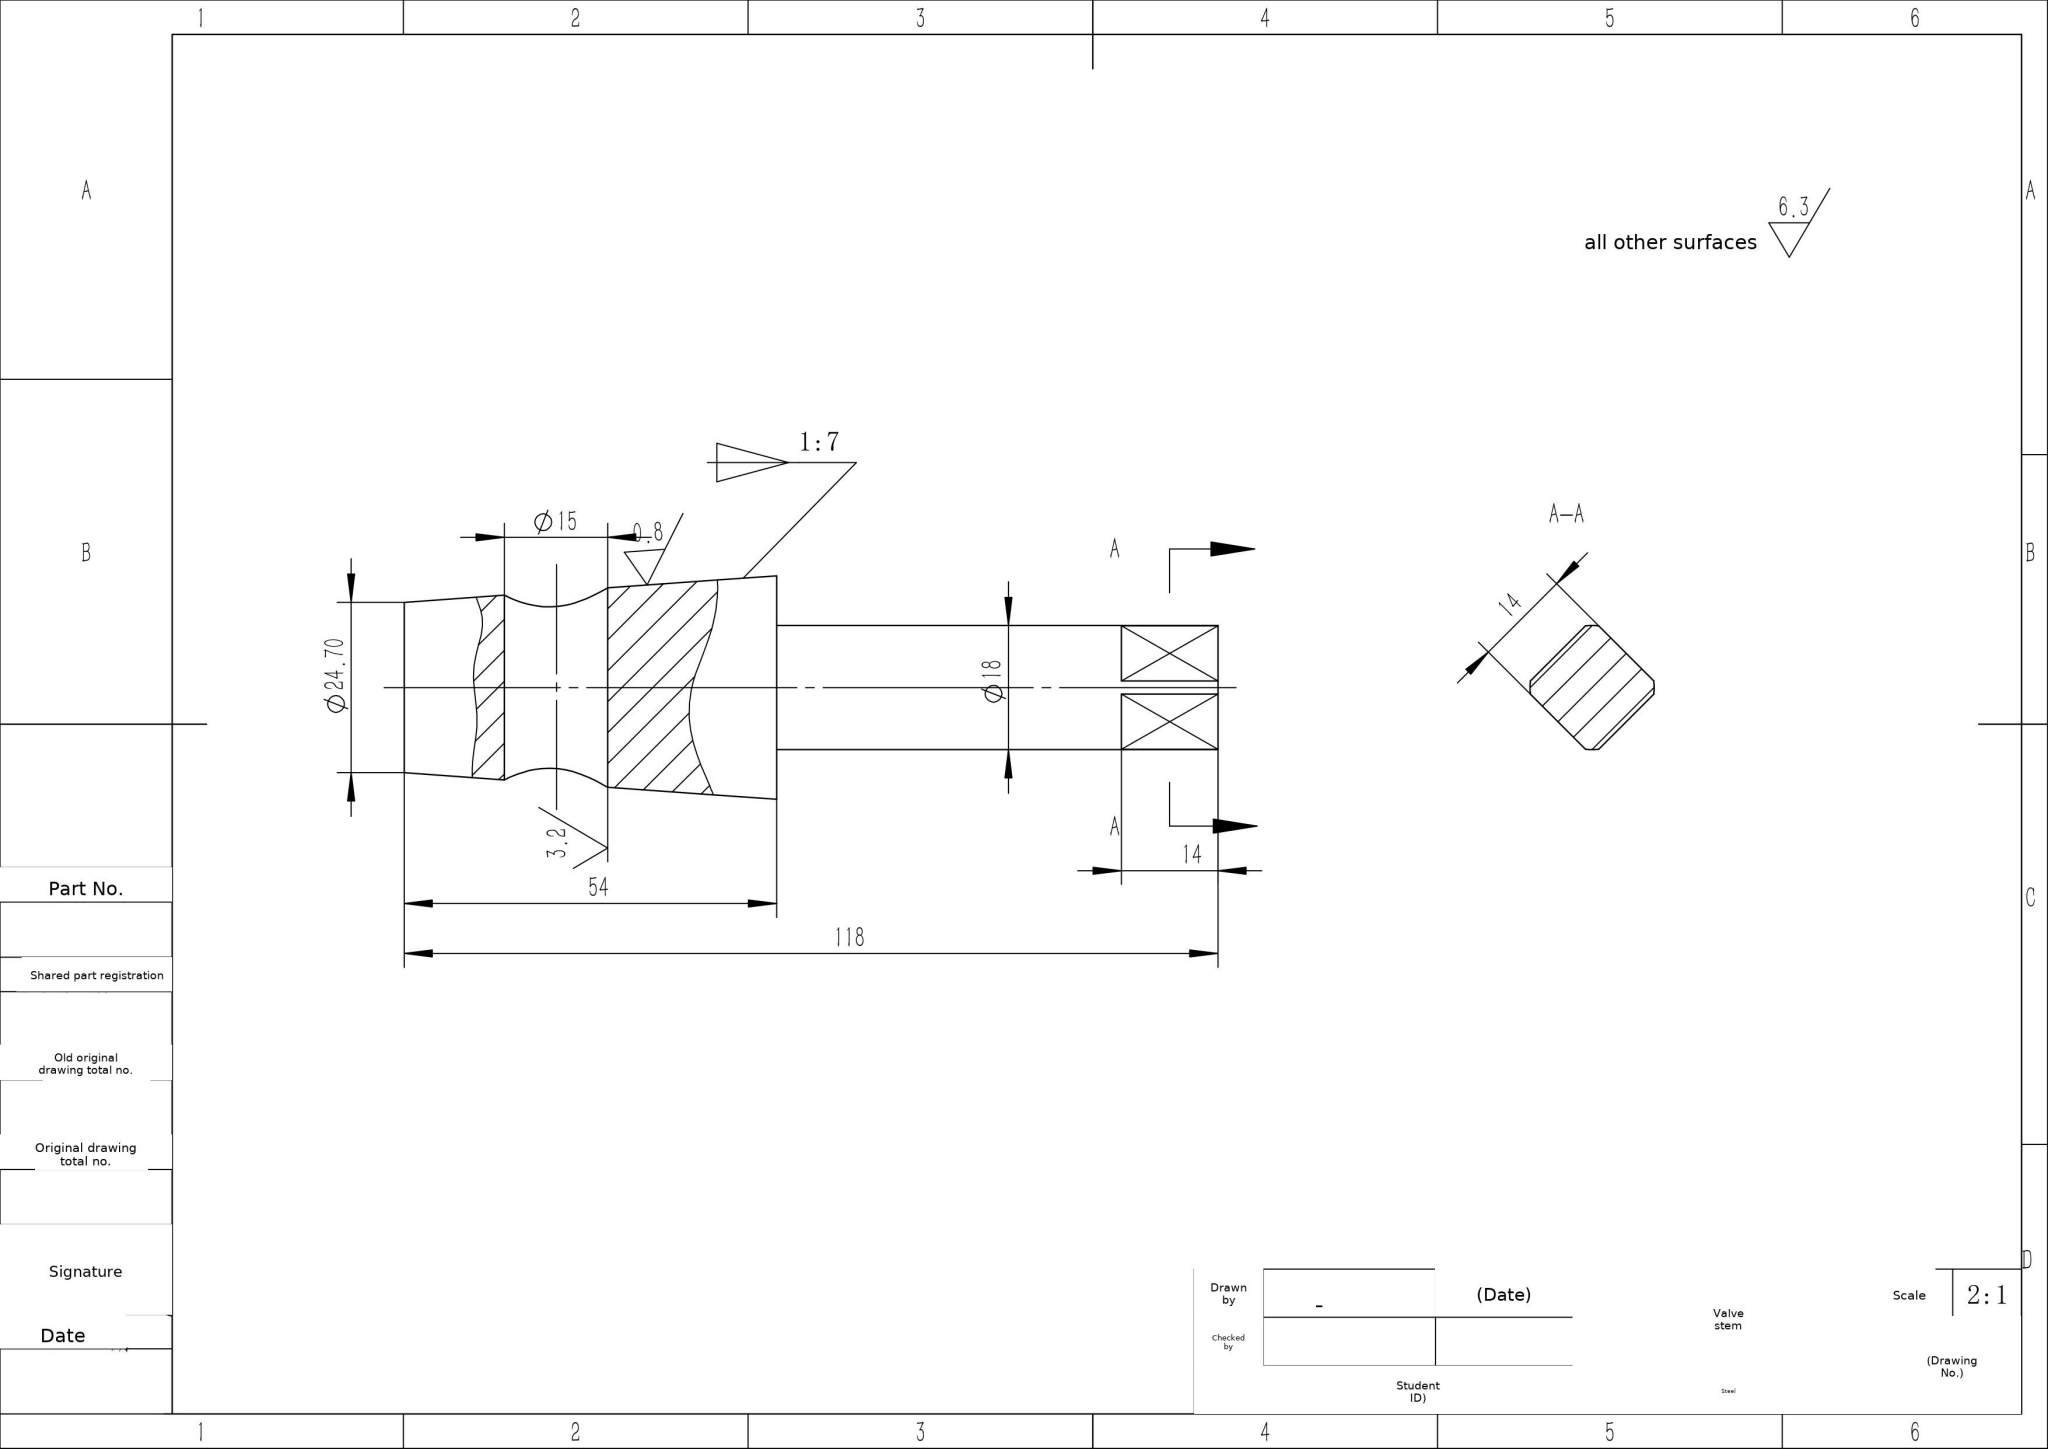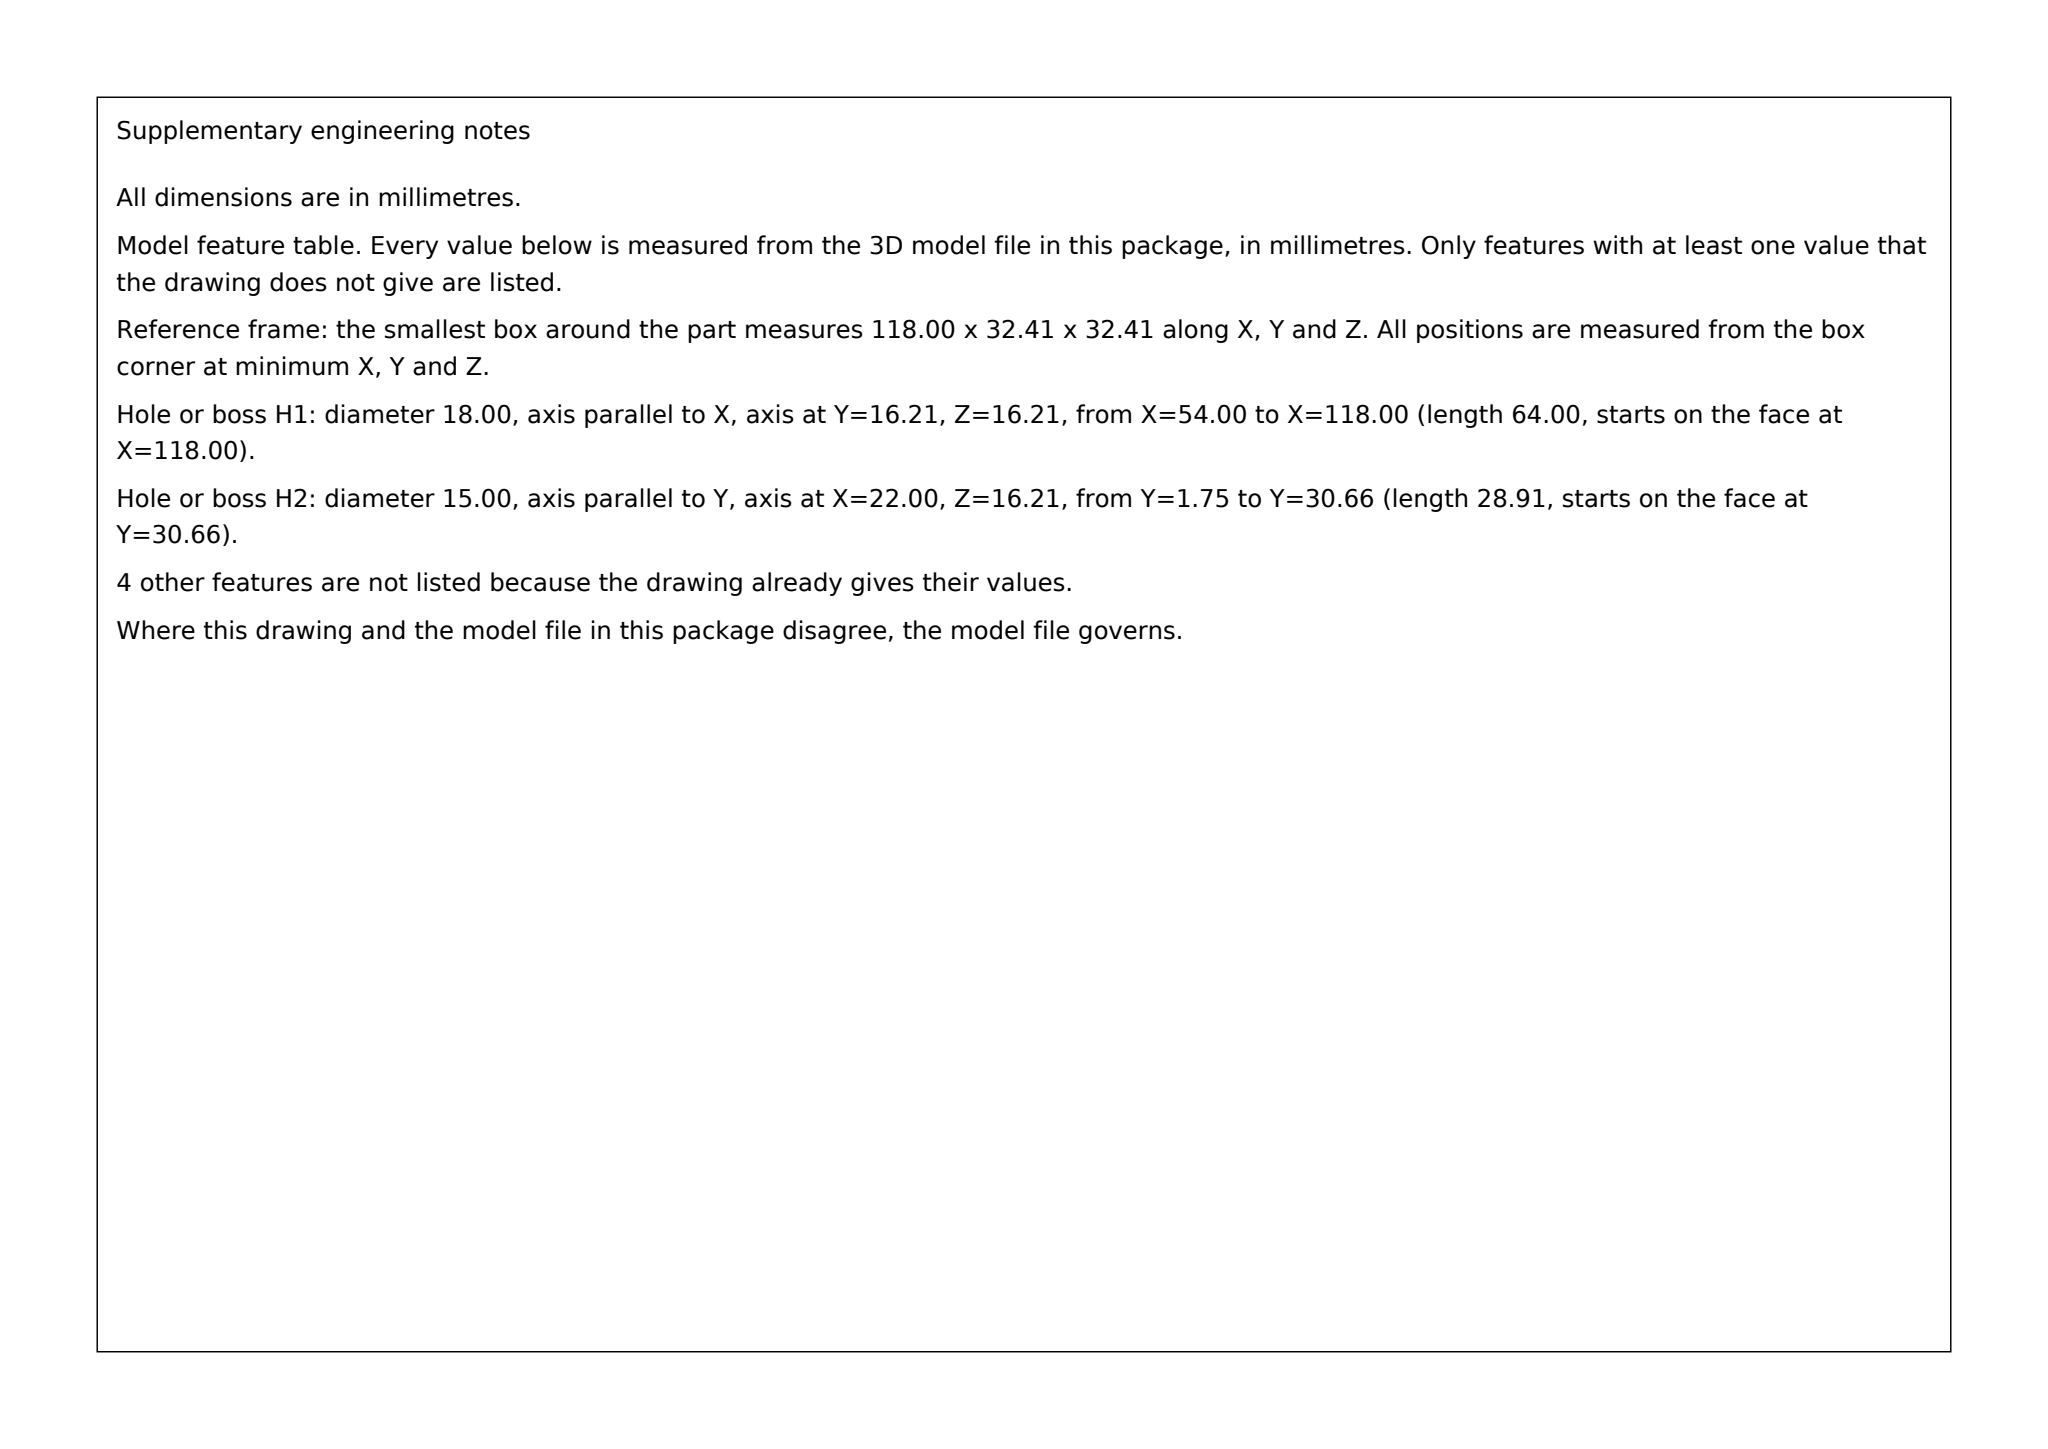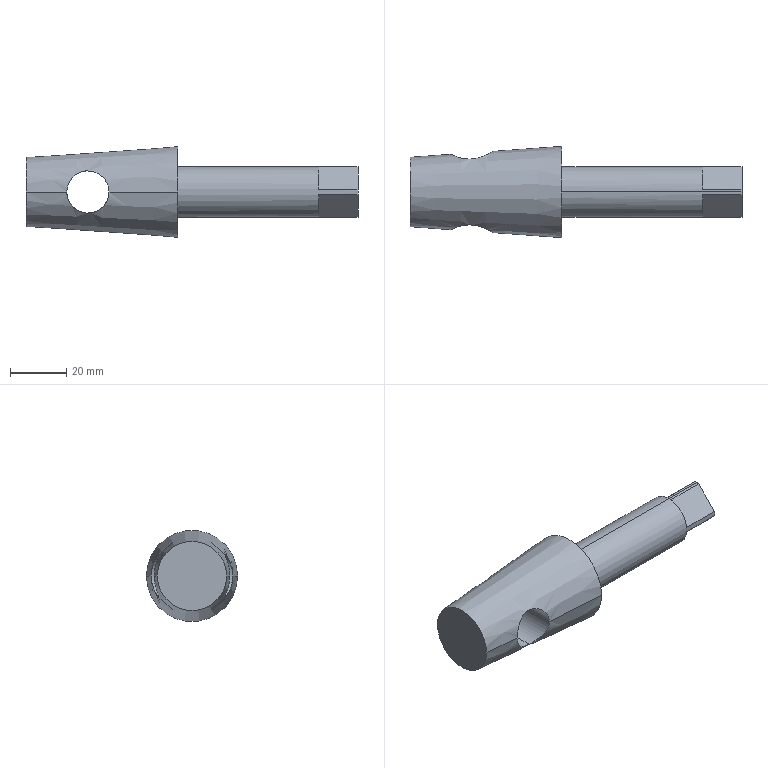Part | SolidWorks | mm | material Steel | 1 solid | 17 faces | box 118 x 32.41 x 32.41 mm | volume 45483 mm3 | plane 11 | cylinder 4 | cone 2 | commonest cylinder face diameters 15 x2 18 x2
build123d program:
from build123d import *

# Parameters (mm, degrees)
SKETCH2_R           = 9
BOSS_EXTRUDE1_DEPTH = 64
SKETCH5_R           = 7.5
CUT_EXTRUDE1_DEPTH  = 32
CUT_EXTRUDE2_DEPTH  = 14


with BuildPart() as part:
    # Sketch2 → Boss-Extrude1 (new body)
    with BuildSketch(Plane(origin=(0, 0, 0), x_dir=(0, 0, -1), z_dir=(1, 0, 0))):
        Circle(SKETCH2_R)
    extrude(amount=BOSS_EXTRUDE1_DEPTH)

    # Sketch3 → Revolve2 (revolve)
    with BuildSketch(Plane.XY, mode=Mode.PRIVATE) as revolve2_sk:
        Polygon((0, 0), (0, 16.207), (-54, 12.35), (-54, 0), align=None)
    revolve(revolve2_sk.sketch.rotate(Axis((-54, 0, 0), (1, 0, 0)), 180), axis=Axis((-54, 0, 0), (1, 0, 0)))

    # Sketch5 → Cut-Extrude1 (cut, symmetric)
    with BuildSketch(Plane(origin=(0, 0, 0), x_dir=(1, 0, 0), z_dir=(0, 1, 0))):
        with Locations(Location((-32, 0, 0), (0, 0, 180))):
            Circle(SKETCH5_R)
    extrude(amount=CUT_EXTRUDE1_DEPTH, both=True, mode=Mode.SUBTRACT)

    # Sketch6 → Cut-Extrude2 (cut)
    with BuildSketch(Plane(origin=(64, 0, 0), x_dir=(0, 0, -1), z_dir=(1, 0, 0))):
        Polygon((-24.042, 0), (0, 24.042), (24.042, 0), (0, -24.042), align=None)
        Polygon((0, -9.899), (9.899, 0), (0, 9.899), (-9.899, 0), align=None, mode=Mode.SUBTRACT)
    extrude(amount=-CUT_EXTRUDE2_DEPTH, mode=Mode.SUBTRACT)


solid = part.part
STEP:
#1=CARTESIAN_POINT('',(-32.,-11.728,-7.5));
#2=VERTEX_POINT('',#1);
#3=CARTESIAN_POINT('',(-39.5,-13.386,0.));
#4=VERTEX_POINT('',#3);
#5=CARTESIAN_POINT('',(-32.,-11.728,-7.5));
#6=CARTESIAN_POINT('',(-32.498,-11.686,-7.5));
#7=CARTESIAN_POINT('',(-32.991,-11.676,-7.451));
#8=CARTESIAN_POINT('',(-33.722,-11.707,-7.304));
#9=CARTESIAN_POINT('',(-33.965,-11.725,-7.242));
#10=CARTESIAN_POINT('',(-34.442,-11.774,-7.096));
#11=CARTESIAN_POINT('',(-34.674,-11.806,-7.011));
#12=CARTESIAN_POINT('',(-35.127,-11.879,-6.821));
#13=CARTESIAN_POINT('',(-35.348,-11.921,-6.716));
#14=CARTESIAN_POINT('',(-35.78,-12.015,-6.483));
#15=CARTESIAN_POINT('',(-35.991,-12.066,-6.355));
#16=CARTESIAN_POINT('',(-36.598,-12.227,-5.945));
#17=CARTESIAN_POINT('',(-36.972,-12.345,-5.636));
#18=CARTESIAN_POINT('',(-37.658,-12.585,-4.947));
#19=CARTESIAN_POINT('',(-37.965,-12.704,-4.572));
#20=CARTESIAN_POINT('',(-38.367,-12.87,-3.971));
#21=CARTESIAN_POINT('',(-38.492,-12.923,-3.764));
#22=CARTESIAN_POINT('',(-38.722,-13.023,-3.335));
#23=CARTESIAN_POINT('',(-38.828,-13.07,-3.112));
#24=CARTESIAN_POINT('',(-39.112,-13.199,-2.432));
#25=CARTESIAN_POINT('',(-39.255,-13.267,-1.964));
#26=CARTESIAN_POINT('',(-39.449,-13.361,-0.9992));
#27=CARTESIAN_POINT('',(-39.5,-13.386,-0.4958));
#28=CARTESIAN_POINT('',(-39.5,-13.386,0.));
#29=B_SPLINE_CURVE_WITH_KNOTS('',3,(#5,#6,#7,#8,#9,#10,#11,#12,#13,#14,#15,#16,#17,#18,#19,#20,#21,#22,#23,#24,#25,#26,#27,#28),.UNSPECIFIED.,.F.,.F.,(4,2,2,2,2,2,2,2,2,2,2,4),(0.04176,0.04324,0.04398,0.04472,0.04547,0.04621,0.04769,0.04917,0.04992,0.05066,0.05214,0.05363),.UNSPECIFIED.);
#30=EDGE_CURVE('',#2,#4,#29,.T.);
#31=ORIENTED_EDGE('',*,*,#30,.F.);
#32=CARTESIAN_POINT('',(-32.,11.728,-7.5));
#33=VERTEX_POINT('',#32);
#34=CARTESIAN_POINT('',(-32.,-32.,-7.5));
#35=DIRECTION('',(0.,1.,0.));
#36=VECTOR('',#35,1000.);
#37=LINE('',#34,#36);
#38=EDGE_CURVE('',#2,#33,#37,.T.);
#39=ORIENTED_EDGE('',*,*,#38,.T.);
#40=CARTESIAN_POINT('',(-39.5,13.386,0.));
#41=VERTEX_POINT('',#40);
#42=CARTESIAN_POINT('',(-39.5,13.386,0.));
#43=CARTESIAN_POINT('',(-39.5,13.386,-0.5028));
#44=CARTESIAN_POINT('',(-39.45,13.361,-0.9965));
#45=CARTESIAN_POINT('',(-39.255,13.267,-1.965));
#46=CARTESIAN_POINT('',(-39.107,13.197,-2.445));
#47=CARTESIAN_POINT('',(-38.729,13.025,-3.349));
#48=CARTESIAN_POINT('',(-38.498,12.923,-3.777));
#49=CARTESIAN_POINT('',(-37.954,12.7,-4.587));
#50=CARTESIAN_POINT('',(-37.644,12.579,-4.963));
#51=CARTESIAN_POINT('',(-37.129,12.4,-5.478));
#52=CARTESIAN_POINT('',(-36.948,12.34,-5.642));
#53=CARTESIAN_POINT('',(-36.573,12.225,-5.949));
#54=CARTESIAN_POINT('',(-36.379,12.169,-6.093));
#55=CARTESIAN_POINT('',(-35.778,12.01,-6.497));
#56=CARTESIAN_POINT('',(-35.348,11.915,-6.73));
#57=CARTESIAN_POINT('',(-34.435,11.767,-7.111));
#58=CARTESIAN_POINT('',(-33.965,11.717,-7.255));
#59=CARTESIAN_POINT('',(-33.24,11.687,-7.401));
#60=CARTESIAN_POINT('',(-32.995,11.684,-7.438));
#61=CARTESIAN_POINT('',(-32.497,11.694,-7.488));
#62=CARTESIAN_POINT('',(-32.247,11.707,-7.5));
#63=CARTESIAN_POINT('',(-32.,11.728,-7.5));
#64=B_SPLINE_CURVE_WITH_KNOTS('',3,(#42,#43,#44,#45,#46,#47,#48,#49,#50,#51,#52,#53,#54,#55,#56,#57,#58,#59,#60,#61,#62,#63),.UNSPECIFIED.,.F.,.F.,(4,2,2,2,2,2,2,2,2,2,4),(0.04154,0.04302,0.04451,0.04599,0.04747,0.04822,0.04896,0.05044,0.05192,0.05267,0.05341),.UNSPECIFIED.);
#65=EDGE_CURVE('',#41,#33,#64,.T.);
#66=ORIENTED_EDGE('',*,*,#65,.F.);
#67=CARTESIAN_POINT('',(-32.,11.728,7.5));
#68=VERTEX_POINT('',#67);
#69=CARTESIAN_POINT('',(-32.,11.728,7.5));
#70=CARTESIAN_POINT('',(-32.499,11.686,7.5));
#71=CARTESIAN_POINT('',(-32.991,11.676,7.451));
#72=CARTESIAN_POINT('',(-33.963,11.717,7.255));
#73=CARTESIAN_POINT('',(-34.446,11.769,7.107));
#74=CARTESIAN_POINT('',(-35.353,11.916,6.727));
#75=CARTESIAN_POINT('',(-35.785,12.011,6.493));
#76=CARTESIAN_POINT('',(-36.597,12.227,5.946));
#77=CARTESIAN_POINT('',(-36.969,12.344,5.639));
#78=CARTESIAN_POINT('',(-37.651,12.582,4.955));
#79=CARTESIAN_POINT('',(-37.963,12.703,4.575));
#80=CARTESIAN_POINT('',(-38.501,12.925,3.771));
#81=CARTESIAN_POINT('',(-38.731,13.026,3.345));
#82=CARTESIAN_POINT('',(-39.015,13.155,2.666));
#83=CARTESIAN_POINT('',(-39.099,13.194,2.431));
#84=CARTESIAN_POINT('',(-39.244,13.262,1.958));
#85=CARTESIAN_POINT('',(-39.304,13.291,1.719));
#86=CARTESIAN_POINT('',(-39.45,13.361,0.9954));
#87=CARTESIAN_POINT('',(-39.5,13.386,0.503));
#88=CARTESIAN_POINT('',(-39.5,13.386,0.));
#89=B_SPLINE_CURVE_WITH_KNOTS('',3,(#69,#70,#71,#72,#73,#74,#75,#76,#77,#78,#79,#80,#81,#82,#83,#84,#85,#86,#87,#88),.UNSPECIFIED.,.F.,.F.,(4,2,2,2,2,2,2,2,2,4),(0.02967,0.03115,0.03264,0.03412,0.0356,0.03709,0.03857,0.03931,0.04006,0.04154),.UNSPECIFIED.);
#90=EDGE_CURVE('',#68,#41,#89,.T.);
#91=ORIENTED_EDGE('',*,*,#90,.F.);
#92=CARTESIAN_POINT('',(-32.,-11.728,7.5));
#93=VERTEX_POINT('',#92);
#94=CARTESIAN_POINT('',(-32.,-32.,7.5));
#95=DIRECTION('',(0.,1.,0.));
#96=VECTOR('',#95,1000.);
#97=LINE('',#94,#96);
#98=EDGE_CURVE('',#93,#68,#97,.T.);
#99=ORIENTED_EDGE('',*,*,#98,.F.);
#100=CARTESIAN_POINT('',(-39.5,-13.386,0.));
#101=CARTESIAN_POINT('',(-39.5,-13.386,0.4967));
#102=CARTESIAN_POINT('',(-39.451,-13.362,0.9892));
#103=CARTESIAN_POINT('',(-39.304,-13.291,1.721));
#104=CARTESIAN_POINT('',(-39.242,-13.262,1.964));
#105=CARTESIAN_POINT('',(-39.098,-13.194,2.436));
#106=CARTESIAN_POINT('',(-39.014,-13.155,2.667));
#107=CARTESIAN_POINT('',(-38.826,-13.069,3.118));
#108=CARTESIAN_POINT('',(-38.721,-13.022,3.338));
#109=CARTESIAN_POINT('',(-38.488,-12.921,3.77));
#110=CARTESIAN_POINT('',(-38.361,-12.867,3.98));
#111=CARTESIAN_POINT('',(-37.955,-12.7,4.585));
#112=CARTESIAN_POINT('',(-37.649,-12.581,4.957));
#113=CARTESIAN_POINT('',(-37.136,-12.403,5.471));
#114=CARTESIAN_POINT('',(-36.955,-12.343,5.636));
#115=CARTESIAN_POINT('',(-36.58,-12.227,5.944));
#116=CARTESIAN_POINT('',(-36.385,-12.171,6.089));
#117=CARTESIAN_POINT('',(-35.784,-12.011,6.494));
#118=CARTESIAN_POINT('',(-35.356,-11.916,6.725));
#119=CARTESIAN_POINT('',(-34.67,-11.805,7.013));
#120=CARTESIAN_POINT('',(-34.436,-11.774,7.098));
#121=CARTESIAN_POINT('',(-33.964,-11.725,7.243));
#122=CARTESIAN_POINT('',(-33.725,-11.707,7.303));
#123=CARTESIAN_POINT('',(-33.241,-11.687,7.401));
#124=CARTESIAN_POINT('',(-32.997,-11.684,7.438));
#125=CARTESIAN_POINT('',(-32.501,-11.694,7.487));
#126=CARTESIAN_POINT('',(-32.249,-11.707,7.5));
#127=CARTESIAN_POINT('',(-32.,-11.728,7.5));
#128=B_SPLINE_CURVE_WITH_KNOTS('',3,(#100,#101,#102,#103,#104,#105,#106,#107,#108,#109,#110,#111,#112,#113,#114,#115,#116,#117,#118,#119,#120,#121,#122,#123,#124,#125,#126,#127),.UNSPECIFIED.,.F.,.F.,(4,2,2,2,2,2,2,2,2,2,2,2,2,4),(0.005728,0.007215,0.007958,0.008701,0.009444,0.01019,0.01167,0.01242,0.01316,0.01465,0.01539,0.01613,0.01688,0.01762),.UNSPECIFIED.);
#129=EDGE_CURVE('',#4,#93,#128,.T.);
#130=ORIENTED_EDGE('',*,*,#129,.F.);
#131=EDGE_LOOP('',(#31,#39,#66,#91,#99,#130));
#132=FACE_OUTER_BOUND('',#131,.T.);
#133=CARTESIAN_POINT('',(-32.,-32.,-0.));
#134=DIRECTION('',(0.,1.,0.));
#135=DIRECTION('',(0.,0.,1.));
#136=AXIS2_PLACEMENT_3D('',#133,#134,#135);
#137=CYLINDRICAL_SURFACE('',#136,7.5);
#138=ADVANCED_FACE('',(#132),#137,.F.);
#139=CARTESIAN_POINT('',(-54.,-12.35,0.));
#140=VERTEX_POINT('',#139);
#141=CARTESIAN_POINT('',(-54.,12.35,0.));
#142=VERTEX_POINT('',#141);
#143=CARTESIAN_POINT('',(-54.,0.,0.));
#144=DIRECTION('',(-1.,0.,0.));
#145=DIRECTION('',(-0.,-1.,0.));
#146=AXIS2_PLACEMENT_3D('',#143,#144,#145);
#147=CIRCLE('',#146,12.35);
#148=EDGE_CURVE('',#140,#142,#147,.T.);
#149=ORIENTED_EDGE('',*,*,#148,.F.);
#150=CARTESIAN_POINT('',(-0.,-16.207,0.));
#151=DIRECTION('',(0.9975,-0.07125,0.));
#152=VECTOR('',#151,1000.);
#153=LINE('',#150,#152);
#154=EDGE_CURVE('',#140,#4,#153,.T.);
#155=ORIENTED_EDGE('',*,*,#154,.T.);
#156=ORIENTED_EDGE('',*,*,#129,.T.);
#157=CARTESIAN_POINT('',(-24.5,-14.457,0.));
#158=VERTEX_POINT('',#157);
#159=CARTESIAN_POINT('',(-32.,-11.728,7.5));
#160=CARTESIAN_POINT('',(-31.494,-11.771,7.5));
#161=CARTESIAN_POINT('',(-30.997,-11.846,7.449));
#162=CARTESIAN_POINT('',(-30.267,-11.999,7.301));
#163=CARTESIAN_POINT('',(-30.025,-12.056,7.239));
#164=CARTESIAN_POINT('',(-29.554,-12.181,7.094));
#165=CARTESIAN_POINT('',(-29.325,-12.248,7.011));
#166=CARTESIAN_POINT('',(-28.878,-12.39,6.824));
#167=CARTESIAN_POINT('',(-28.66,-12.465,6.719));
#168=CARTESIAN_POINT('',(-28.233,-12.62,6.49));
#169=CARTESIAN_POINT('',(-28.025,-12.701,6.365));
#170=CARTESIAN_POINT('',(-27.427,-12.944,5.964));
#171=CARTESIAN_POINT('',(-27.058,-13.109,5.662));
#172=CARTESIAN_POINT('',(-26.377,-13.432,4.986));
#173=CARTESIAN_POINT('',(-26.065,-13.591,4.61));
#174=CARTESIAN_POINT('',(-25.523,-13.876,3.811));
#175=CARTESIAN_POINT('',(-25.289,-14.005,3.385));
#176=CARTESIAN_POINT('',(-24.999,-14.168,2.702));
#177=CARTESIAN_POINT('',(-24.912,-14.218,2.465));
#178=CARTESIAN_POINT('',(-24.764,-14.303,1.988));
#179=CARTESIAN_POINT('',(-24.702,-14.339,1.746));
#180=CARTESIAN_POINT('',(-24.552,-14.426,1.013));
#181=CARTESIAN_POINT('',(-24.5,-14.457,0.5114));
#182=CARTESIAN_POINT('',(-24.5,-14.457,0.));
#183=B_SPLINE_CURVE_WITH_KNOTS('',3,(#159,#160,#161,#162,#163,#164,#165,#166,#167,#168,#169,#170,#171,#172,#173,#174,#175,#176,#177,#178,#179,#180,#181,#182),.UNSPECIFIED.,.F.,.F.,(4,2,2,2,2,2,2,2,2,2,2,4),(0.01762,0.01913,0.01988,0.02064,0.02139,0.02215,0.02366,0.02517,0.02668,0.02744,0.02819,0.0297),.UNSPECIFIED.);
#184=EDGE_CURVE('',#93,#158,#183,.T.);
#185=ORIENTED_EDGE('',*,*,#184,.T.);
#186=CARTESIAN_POINT('',(-0.,-16.207,0.));
#187=VERTEX_POINT('',#186);
#188=CARTESIAN_POINT('',(-0.,-16.207,0.));
#189=DIRECTION('',(0.9975,-0.07125,0.));
#190=VECTOR('',#189,1000.);
#191=LINE('',#188,#190);
#192=EDGE_CURVE('',#158,#187,#191,.T.);
#193=ORIENTED_EDGE('',*,*,#192,.T.);
#194=CARTESIAN_POINT('',(-0.,16.207,0.));
#195=VERTEX_POINT('',#194);
#196=CARTESIAN_POINT('',(-0.,0.,0.));
#197=DIRECTION('',(-1.,0.,0.));
#198=DIRECTION('',(-0.,-1.,0.));
#199=AXIS2_PLACEMENT_3D('',#196,#197,#198);
#200=CIRCLE('',#199,16.207);
#201=EDGE_CURVE('',#187,#195,#200,.T.);
#202=ORIENTED_EDGE('',*,*,#201,.T.);
#203=CARTESIAN_POINT('',(-24.5,14.457,-0.));
#204=VERTEX_POINT('',#203);
#205=CARTESIAN_POINT('',(-0.,16.207,0.));
#206=DIRECTION('',(0.9975,0.07125,0.));
#207=VECTOR('',#206,1000.);
#208=LINE('',#205,#207);
#209=EDGE_CURVE('',#204,#195,#208,.T.);
#210=ORIENTED_EDGE('',*,*,#209,.F.);
#211=CARTESIAN_POINT('',(-24.5,14.457,-0.));
#212=CARTESIAN_POINT('',(-24.5,14.457,0.507));
#213=CARTESIAN_POINT('',(-24.551,14.427,1.007));
#214=CARTESIAN_POINT('',(-24.702,14.339,1.747));
#215=CARTESIAN_POINT('',(-24.765,14.302,1.994));
#216=CARTESIAN_POINT('',(-24.914,14.216,2.471));
#217=CARTESIAN_POINT('',(-25.,14.168,2.704));
#218=CARTESIAN_POINT('',(-25.193,14.059,3.158));
#219=CARTESIAN_POINT('',(-25.3,14.,3.379));
#220=CARTESIAN_POINT('',(-25.536,13.871,3.811));
#221=CARTESIAN_POINT('',(-25.664,13.802,4.021));
#222=CARTESIAN_POINT('',(-26.075,13.586,4.624));
#223=CARTESIAN_POINT('',(-26.382,13.43,4.992));
#224=CARTESIAN_POINT('',(-26.895,13.186,5.5));
#225=CARTESIAN_POINT('',(-27.075,13.103,5.662));
#226=CARTESIAN_POINT('',(-27.447,12.939,5.965));
#227=CARTESIAN_POINT('',(-27.639,12.857,6.107));
#228=CARTESIAN_POINT('',(-28.235,12.616,6.504));
#229=CARTESIAN_POINT('',(-28.657,12.46,6.732));
#230=CARTESIAN_POINT('',(-29.561,12.174,7.109));
#231=CARTESIAN_POINT('',(-30.029,12.048,7.253));
#232=CARTESIAN_POINT('',(-30.751,11.898,7.399));
#233=CARTESIAN_POINT('',(-30.995,11.854,7.437));
#234=CARTESIAN_POINT('',(-31.492,11.78,7.487));
#235=CARTESIAN_POINT('',(-31.746,11.75,7.5));
#236=CARTESIAN_POINT('',(-32.,11.728,7.5));
#237=B_SPLINE_CURVE_WITH_KNOTS('',3,(#211,#212,#213,#214,#215,#216,#217,#218,#219,#220,#221,#222,#223,#224,#225,#226,#227,#228,#229,#230,#231,#232,#233,#234,#235,#236),.UNSPECIFIED.,.F.,.F.,(4,2,2,2,2,2,2,2,2,2,2,2,4),(0.01758,0.01909,0.01985,0.0206,0.02136,0.02211,0.02362,0.02438,0.02514,0.02665,0.02816,0.02891,0.02967),.UNSPECIFIED.);
#238=EDGE_CURVE('',#204,#68,#237,.T.);
#239=ORIENTED_EDGE('',*,*,#238,.T.);
#240=ORIENTED_EDGE('',*,*,#90,.T.);
#241=CARTESIAN_POINT('',(-0.,16.207,0.));
#242=DIRECTION('',(0.9975,0.07125,0.));
#243=VECTOR('',#242,1000.);
#244=LINE('',#241,#243);
#245=EDGE_CURVE('',#142,#41,#244,.T.);
#246=ORIENTED_EDGE('',*,*,#245,.F.);
#247=EDGE_LOOP('',(#149,#155,#156,#185,#193,#202,#210,#239,#240,#246));
#248=FACE_OUTER_BOUND('',#247,.T.);
#249=CARTESIAN_POINT('',(-0.,0.,0.));
#250=DIRECTION('',(1.,-0.,0.));
#251=DIRECTION('',(0.,1.,0.));
#252=AXIS2_PLACEMENT_3D('',#249,#250,#251);
#253=CONICAL_SURFACE('',#252,16.207,0.07131);
#254=ADVANCED_FACE('',(#248),#253,.T.);
#255=CARTESIAN_POINT('',(64.,0.,-9.));
#256=VERTEX_POINT('',#255);
#257=CARTESIAN_POINT('',(64.,0.9497,-8.95));
#258=VERTEX_POINT('',#257);
#259=CARTESIAN_POINT('',(64.,0.,0.));
#260=DIRECTION('',(1.,0.,0.));
#261=DIRECTION('',(0.,0.,-1.));
#262=AXIS2_PLACEMENT_3D('',#259,#260,#261);
#263=CIRCLE('',#262,9.);
#264=EDGE_CURVE('',#256,#258,#263,.T.);
#265=ORIENTED_EDGE('',*,*,#264,.F.);
#266=CARTESIAN_POINT('',(0.,0.,-9.));
#267=VERTEX_POINT('',#266);
#268=CARTESIAN_POINT('',(64.,0.,-9.));
#269=DIRECTION('',(-1.,0.,0.));
#270=VECTOR('',#269,1000.);
#271=LINE('',#268,#270);
#272=EDGE_CURVE('',#256,#267,#271,.T.);
#273=ORIENTED_EDGE('',*,*,#272,.T.);
#274=CARTESIAN_POINT('',(0.,0.,9.));
#275=VERTEX_POINT('',#274);
#276=CARTESIAN_POINT('',(0.,0.,0.));
#277=DIRECTION('',(1.,0.,0.));
#278=DIRECTION('',(0.,0.,-1.));
#279=AXIS2_PLACEMENT_3D('',#276,#277,#278);
#280=CIRCLE('',#279,9.);
#281=EDGE_CURVE('',#267,#275,#280,.T.);
#282=ORIENTED_EDGE('',*,*,#281,.T.);
#283=CARTESIAN_POINT('',(64.,0.,9.));
#284=VERTEX_POINT('',#283);
#285=CARTESIAN_POINT('',(64.,0.,9.));
#286=DIRECTION('',(-1.,0.,0.));
#287=VECTOR('',#286,1000.);
#288=LINE('',#285,#287);
#289=EDGE_CURVE('',#284,#275,#288,.T.);
#290=ORIENTED_EDGE('',*,*,#289,.F.);
#291=CARTESIAN_POINT('',(64.,0.9497,8.95));
#292=VERTEX_POINT('',#291);
#293=CARTESIAN_POINT('',(64.,0.,0.));
#294=DIRECTION('',(1.,0.,0.));
#295=DIRECTION('',(0.,0.,-1.));
#296=AXIS2_PLACEMENT_3D('',#293,#294,#295);
#297=CIRCLE('',#296,9.);
#298=EDGE_CURVE('',#292,#284,#297,.T.);
#299=ORIENTED_EDGE('',*,*,#298,.F.);
#300=CARTESIAN_POINT('',(50.,0.9497,8.95));
#301=VERTEX_POINT('',#300);
#302=CARTESIAN_POINT('',(64.,0.9497,8.95));
#303=DIRECTION('',(1.,0.,0.));
#304=VECTOR('',#303,1000.);
#305=LINE('',#302,#304);
#306=EDGE_CURVE('',#301,#292,#305,.T.);
#307=ORIENTED_EDGE('',*,*,#306,.F.);
#308=CARTESIAN_POINT('',(50.,8.95,0.9497));
#309=VERTEX_POINT('',#308);
#310=CARTESIAN_POINT('',(50.,0.,0.));
#311=DIRECTION('',(-1.,0.,0.));
#312=DIRECTION('',(0.,0.,1.));
#313=AXIS2_PLACEMENT_3D('',#310,#311,#312);
#314=CIRCLE('',#313,9.);
#315=EDGE_CURVE('',#301,#309,#314,.T.);
#316=ORIENTED_EDGE('',*,*,#315,.T.);
#317=CARTESIAN_POINT('',(64.,8.95,0.9497));
#318=VERTEX_POINT('',#317);
#319=CARTESIAN_POINT('',(64.,8.95,0.9497));
#320=DIRECTION('',(-1.,0.,0.));
#321=VECTOR('',#320,1000.);
#322=LINE('',#319,#321);
#323=EDGE_CURVE('',#318,#309,#322,.T.);
#324=ORIENTED_EDGE('',*,*,#323,.F.);
#325=CARTESIAN_POINT('',(64.,8.95,-0.9497));
#326=VERTEX_POINT('',#325);
#327=CARTESIAN_POINT('',(64.,0.,0.));
#328=DIRECTION('',(1.,0.,0.));
#329=DIRECTION('',(0.,0.,-1.));
#330=AXIS2_PLACEMENT_3D('',#327,#328,#329);
#331=CIRCLE('',#330,9.);
#332=EDGE_CURVE('',#326,#318,#331,.T.);
#333=ORIENTED_EDGE('',*,*,#332,.F.);
#334=CARTESIAN_POINT('',(50.,8.95,-0.9497));
#335=VERTEX_POINT('',#334);
#336=CARTESIAN_POINT('',(64.,8.95,-0.9497));
#337=DIRECTION('',(1.,0.,0.));
#338=VECTOR('',#337,1000.);
#339=LINE('',#336,#338);
#340=EDGE_CURVE('',#335,#326,#339,.T.);
#341=ORIENTED_EDGE('',*,*,#340,.F.);
#342=CARTESIAN_POINT('',(50.,0.9497,-8.95));
#343=VERTEX_POINT('',#342);
#344=CARTESIAN_POINT('',(50.,0.,0.));
#345=DIRECTION('',(-1.,0.,0.));
#346=DIRECTION('',(0.,0.,1.));
#347=AXIS2_PLACEMENT_3D('',#344,#345,#346);
#348=CIRCLE('',#347,9.);
#349=EDGE_CURVE('',#335,#343,#348,.T.);
#350=ORIENTED_EDGE('',*,*,#349,.T.);
#351=CARTESIAN_POINT('',(64.,0.9497,-8.95));
#352=DIRECTION('',(-1.,0.,0.));
#353=VECTOR('',#352,1000.);
#354=LINE('',#351,#353);
#355=EDGE_CURVE('',#258,#343,#354,.T.);
#356=ORIENTED_EDGE('',*,*,#355,.F.);
#357=EDGE_LOOP('',(#265,#273,#282,#290,#299,#307,#316,#324,#333,#341,#350,#356));
#358=FACE_OUTER_BOUND('',#357,.T.);
#359=CARTESIAN_POINT('',(64.,0.,0.));
#360=DIRECTION('',(-1.,0.,0.));
#361=DIRECTION('',(0.,0.,1.));
#362=AXIS2_PLACEMENT_3D('',#359,#360,#361);
#363=CYLINDRICAL_SURFACE('',#362,9.);
#364=ADVANCED_FACE('',(#358),#363,.T.);
#365=ORIENTED_EDGE('',*,*,#272,.F.);
#366=CARTESIAN_POINT('',(64.,-0.9497,-8.95));
#367=VERTEX_POINT('',#366);
#368=CARTESIAN_POINT('',(64.,0.,0.));
#369=DIRECTION('',(1.,0.,0.));
#370=DIRECTION('',(0.,0.,-1.));
#371=AXIS2_PLACEMENT_3D('',#368,#369,#370);
#372=CIRCLE('',#371,9.);
#373=EDGE_CURVE('',#367,#256,#372,.T.);
#374=ORIENTED_EDGE('',*,*,#373,.F.);
#375=CARTESIAN_POINT('',(50.,-0.9497,-8.95));
#376=VERTEX_POINT('',#375);
#377=CARTESIAN_POINT('',(64.,-0.9497,-8.95));
#378=DIRECTION('',(1.,0.,0.));
#379=VECTOR('',#378,1000.);
#380=LINE('',#377,#379);
#381=EDGE_CURVE('',#376,#367,#380,.T.);
#382=ORIENTED_EDGE('',*,*,#381,.F.);
#383=CARTESIAN_POINT('',(50.,-8.95,-0.9497));
#384=VERTEX_POINT('',#383);
#385=CARTESIAN_POINT('',(50.,0.,0.));
#386=DIRECTION('',(-1.,0.,0.));
#387=DIRECTION('',(0.,0.,1.));
#388=AXIS2_PLACEMENT_3D('',#385,#386,#387);
#389=CIRCLE('',#388,9.);
#390=EDGE_CURVE('',#376,#384,#389,.T.);
#391=ORIENTED_EDGE('',*,*,#390,.T.);
#392=CARTESIAN_POINT('',(64.,-8.95,-0.9497));
#393=VERTEX_POINT('',#392);
#394=CARTESIAN_POINT('',(64.,-8.95,-0.9497));
#395=DIRECTION('',(-1.,0.,0.));
#396=VECTOR('',#395,1000.);
#397=LINE('',#394,#396);
#398=EDGE_CURVE('',#393,#384,#397,.T.);
#399=ORIENTED_EDGE('',*,*,#398,.F.);
#400=CARTESIAN_POINT('',(64.,-8.95,0.9497));
#401=VERTEX_POINT('',#400);
#402=CARTESIAN_POINT('',(64.,0.,0.));
#403=DIRECTION('',(1.,0.,0.));
#404=DIRECTION('',(0.,0.,-1.));
#405=AXIS2_PLACEMENT_3D('',#402,#403,#404);
#406=CIRCLE('',#405,9.);
#407=EDGE_CURVE('',#401,#393,#406,.T.);
#408=ORIENTED_EDGE('',*,*,#407,.F.);
#409=CARTESIAN_POINT('',(50.,-8.95,0.9497));
#410=VERTEX_POINT('',#409);
#411=CARTESIAN_POINT('',(64.,-8.95,0.9497));
#412=DIRECTION('',(1.,0.,0.));
#413=VECTOR('',#412,1000.);
#414=LINE('',#411,#413);
#415=EDGE_CURVE('',#410,#401,#414,.T.);
#416=ORIENTED_EDGE('',*,*,#415,.F.);
#417=CARTESIAN_POINT('',(50.,-0.9497,8.95));
#418=VERTEX_POINT('',#417);
#419=CARTESIAN_POINT('',(50.,0.,0.));
#420=DIRECTION('',(-1.,0.,0.));
#421=DIRECTION('',(0.,0.,1.));
#422=AXIS2_PLACEMENT_3D('',#419,#420,#421);
#423=CIRCLE('',#422,9.);
#424=EDGE_CURVE('',#410,#418,#423,.T.);
#425=ORIENTED_EDGE('',*,*,#424,.T.);
#426=CARTESIAN_POINT('',(64.,-0.9497,8.95));
#427=VERTEX_POINT('',#426);
#428=CARTESIAN_POINT('',(64.,-0.9497,8.95));
#429=DIRECTION('',(-1.,0.,0.));
#430=VECTOR('',#429,1000.);
#431=LINE('',#428,#430);
#432=EDGE_CURVE('',#427,#418,#431,.T.);
#433=ORIENTED_EDGE('',*,*,#432,.F.);
#434=CARTESIAN_POINT('',(64.,0.,0.));
#435=DIRECTION('',(1.,0.,0.));
#436=DIRECTION('',(0.,0.,-1.));
#437=AXIS2_PLACEMENT_3D('',#434,#435,#436);
#438=CIRCLE('',#437,9.);
#439=EDGE_CURVE('',#284,#427,#438,.T.);
#440=ORIENTED_EDGE('',*,*,#439,.F.);
#441=ORIENTED_EDGE('',*,*,#289,.T.);
#442=CARTESIAN_POINT('',(0.,0.,0.));
#443=DIRECTION('',(1.,0.,0.));
#444=DIRECTION('',(0.,0.,-1.));
#445=AXIS2_PLACEMENT_3D('',#442,#443,#444);
#446=CIRCLE('',#445,9.);
#447=EDGE_CURVE('',#275,#267,#446,.T.);
#448=ORIENTED_EDGE('',*,*,#447,.T.);
#449=EDGE_LOOP('',(#365,#374,#382,#391,#399,#408,#416,#425,#433,#440,#441,#448));
#450=FACE_OUTER_BOUND('',#449,.T.);
#451=CARTESIAN_POINT('',(64.,0.,0.));
#452=DIRECTION('',(-1.,0.,0.));
#453=DIRECTION('',(0.,0.,1.));
#454=AXIS2_PLACEMENT_3D('',#451,#452,#453);
#455=CYLINDRICAL_SURFACE('',#454,9.);
#456=ADVANCED_FACE('',(#450),#455,.T.);
#457=ORIENTED_EDGE('',*,*,#373,.T.);
#458=ORIENTED_EDGE('',*,*,#264,.T.);
#459=CARTESIAN_POINT('',(64.,4.95,-4.95));
#460=DIRECTION('',(0.,0.7071,0.7071));
#461=VECTOR('',#460,1000.);
#462=LINE('',#459,#461);
#463=EDGE_CURVE('',#258,#326,#462,.T.);
#464=ORIENTED_EDGE('',*,*,#463,.T.);
#465=ORIENTED_EDGE('',*,*,#332,.T.);
#466=CARTESIAN_POINT('',(64.,4.95,4.95));
#467=DIRECTION('',(0.,-0.7071,0.7071));
#468=VECTOR('',#467,1000.);
#469=LINE('',#466,#468);
#470=EDGE_CURVE('',#318,#292,#469,.T.);
#471=ORIENTED_EDGE('',*,*,#470,.T.);
#472=ORIENTED_EDGE('',*,*,#298,.T.);
#473=ORIENTED_EDGE('',*,*,#439,.T.);
#474=CARTESIAN_POINT('',(64.,-4.95,4.95));
#475=DIRECTION('',(0.,-0.7071,-0.7071));
#476=VECTOR('',#475,1000.);
#477=LINE('',#474,#476);
#478=EDGE_CURVE('',#427,#401,#477,.T.);
#479=ORIENTED_EDGE('',*,*,#478,.T.);
#480=ORIENTED_EDGE('',*,*,#407,.T.);
#481=CARTESIAN_POINT('',(64.,-4.95,-4.95));
#482=DIRECTION('',(0.,0.7071,-0.7071));
#483=VECTOR('',#482,1000.);
#484=LINE('',#481,#483);
#485=EDGE_CURVE('',#393,#367,#484,.T.);
#486=ORIENTED_EDGE('',*,*,#485,.T.);
#487=EDGE_LOOP('',(#457,#458,#464,#465,#471,#472,#473,#479,#480,#486));
#488=FACE_OUTER_BOUND('',#487,.T.);
#489=CARTESIAN_POINT('',(64.,0.,0.));
#490=DIRECTION('',(1.,0.,0.));
#491=DIRECTION('',(0.,0.,-1.));
#492=AXIS2_PLACEMENT_3D('',#489,#490,#491);
#493=PLANE('',#492);
#494=ADVANCED_FACE('',(#488),#493,.T.);
#495=ORIENTED_EDGE('',*,*,#447,.F.);
#496=ORIENTED_EDGE('',*,*,#281,.F.);
#497=EDGE_LOOP('',(#495,#496));
#498=FACE_BOUND('',#497,.T.);
#499=CARTESIAN_POINT('',(-0.,0.,0.));
#500=DIRECTION('',(-1.,0.,0.));
#501=DIRECTION('',(-0.,-1.,0.));
#502=AXIS2_PLACEMENT_3D('',#499,#500,#501);
#503=CIRCLE('',#502,16.207);
#504=EDGE_CURVE('',#195,#187,#503,.T.);
#505=ORIENTED_EDGE('',*,*,#504,.F.);
#506=ORIENTED_EDGE('',*,*,#201,.F.);
#507=EDGE_LOOP('',(#505,#506));
#508=FACE_OUTER_BOUND('',#507,.T.);
#509=CARTESIAN_POINT('',(-0.,0.,0.));
#510=DIRECTION('',(-1.,0.,0.));
#511=DIRECTION('',(-0.,-1.,0.));
#512=AXIS2_PLACEMENT_3D('',#509,#510,#511);
#513=PLANE('',#512);
#514=ADVANCED_FACE('',(#498,#508),#513,.F.);
#515=ORIENTED_EDGE('',*,*,#154,.F.);
#516=CARTESIAN_POINT('',(-54.,0.,0.));
#517=DIRECTION('',(-1.,0.,0.));
#518=DIRECTION('',(-0.,-1.,0.));
#519=AXIS2_PLACEMENT_3D('',#516,#517,#518);
#520=CIRCLE('',#519,12.35);
#521=EDGE_CURVE('',#142,#140,#520,.T.);
#522=ORIENTED_EDGE('',*,*,#521,.F.);
#523=ORIENTED_EDGE('',*,*,#245,.T.);
#524=ORIENTED_EDGE('',*,*,#65,.T.);
#525=CARTESIAN_POINT('',(-32.,11.728,-7.5));
#526=CARTESIAN_POINT('',(-31.496,11.771,-7.5));
#527=CARTESIAN_POINT('',(-31.,11.846,-7.45));
#528=CARTESIAN_POINT('',(-30.02,12.05,-7.251));
#529=CARTESIAN_POINT('',(-29.551,12.177,-7.105));
#530=CARTESIAN_POINT('',(-28.655,12.461,-6.73));
#531=CARTESIAN_POINT('',(-28.225,12.62,-6.498));
#532=CARTESIAN_POINT('',(-27.429,12.943,-5.965));
#533=CARTESIAN_POINT('',(-27.06,13.108,-5.664));
#534=CARTESIAN_POINT('',(-26.547,13.352,-5.155));
#535=CARTESIAN_POINT('',(-26.383,13.432,-4.975));
#536=CARTESIAN_POINT('',(-26.075,13.587,-4.605));
#537=CARTESIAN_POINT('',(-25.931,13.661,-4.413));
#538=CARTESIAN_POINT('',(-25.525,13.875,-3.815));
#539=CARTESIAN_POINT('',(-25.29,14.004,-3.388));
#540=CARTESIAN_POINT('',(-24.9,14.224,-2.469));
#541=CARTESIAN_POINT('',(-24.753,14.309,-1.995));
#542=CARTESIAN_POINT('',(-24.603,14.397,-1.262));
#543=CARTESIAN_POINT('',(-24.565,14.419,-1.014));
#544=CARTESIAN_POINT('',(-24.513,14.449,-0.5106));
#545=CARTESIAN_POINT('',(-24.5,14.457,-0.2537));
#546=CARTESIAN_POINT('',(-24.5,14.457,-0.));
#547=B_SPLINE_CURVE_WITH_KNOTS('',3,(#525,#526,#527,#528,#529,#530,#531,#532,#533,#534,#535,#536,#537,#538,#539,#540,#541,#542,#543,#544,#545,#546),.UNSPECIFIED.,.F.,.F.,(4,2,2,2,2,2,2,2,2,2,4),(0.005488,0.007,0.008512,0.01002,0.01154,0.01229,0.01305,0.01456,0.01607,0.01683,0.01758),.UNSPECIFIED.);
#548=EDGE_CURVE('',#33,#204,#547,.T.);
#549=ORIENTED_EDGE('',*,*,#548,.T.);
#550=ORIENTED_EDGE('',*,*,#209,.T.);
#551=ORIENTED_EDGE('',*,*,#504,.T.);
#552=ORIENTED_EDGE('',*,*,#192,.F.);
#553=CARTESIAN_POINT('',(-24.5,-14.457,0.));
#554=CARTESIAN_POINT('',(-24.5,-14.457,-0.5104));
#555=CARTESIAN_POINT('',(-24.552,-14.427,-1.011));
#556=CARTESIAN_POINT('',(-24.752,-14.309,-1.993));
#557=CARTESIAN_POINT('',(-24.904,-14.222,-2.477));
#558=CARTESIAN_POINT('',(-25.289,-14.005,-3.385));
#559=CARTESIAN_POINT('',(-25.525,-13.875,-3.816));
#560=CARTESIAN_POINT('',(-26.074,-13.586,-4.623));
#561=CARTESIAN_POINT('',(-26.382,-13.43,-4.991));
#562=CARTESIAN_POINT('',(-27.061,-13.107,-5.665));
#563=CARTESIAN_POINT('',(-27.437,-12.939,-5.972));
#564=CARTESIAN_POINT('',(-28.232,-12.617,-6.502));
#565=CARTESIAN_POINT('',(-28.653,-12.462,-6.729));
#566=CARTESIAN_POINT('',(-29.325,-12.249,-7.011));
#567=CARTESIAN_POINT('',(-29.556,-12.181,-7.095));
#568=CARTESIAN_POINT('',(-30.027,-12.056,-7.24));
#569=CARTESIAN_POINT('',(-30.266,-11.999,-7.301));
#570=CARTESIAN_POINT('',(-30.749,-11.898,-7.399));
#571=CARTESIAN_POINT('',(-30.995,-11.854,-7.437));
#572=CARTESIAN_POINT('',(-31.492,-11.78,-7.487));
#573=CARTESIAN_POINT('',(-31.747,-11.75,-7.5));
#574=CARTESIAN_POINT('',(-32.,-11.728,-7.5));
#575=B_SPLINE_CURVE_WITH_KNOTS('',3,(#553,#554,#555,#556,#557,#558,#559,#560,#561,#562,#563,#564,#565,#566,#567,#568,#569,#570,#571,#572,#573,#574),.UNSPECIFIED.,.F.,.F.,(4,2,2,2,2,2,2,2,2,2,4),(0.0297,0.03121,0.03271,0.03422,0.03573,0.03724,0.03874,0.0395,0.04025,0.041,0.04176),.UNSPECIFIED.);
#576=EDGE_CURVE('',#158,#2,#575,.T.);
#577=ORIENTED_EDGE('',*,*,#576,.T.);
#578=ORIENTED_EDGE('',*,*,#30,.T.);
#579=EDGE_LOOP('',(#515,#522,#523,#524,#549,#550,#551,#552,#577,#578));
#580=FACE_OUTER_BOUND('',#579,.T.);
#581=CARTESIAN_POINT('',(-0.,0.,0.));
#582=DIRECTION('',(1.,-0.,0.));
#583=DIRECTION('',(0.,1.,0.));
#584=AXIS2_PLACEMENT_3D('',#581,#582,#583);
#585=CONICAL_SURFACE('',#584,16.207,0.07131);
#586=ADVANCED_FACE('',(#580),#585,.T.);
#587=ORIENTED_EDGE('',*,*,#521,.T.);
#588=ORIENTED_EDGE('',*,*,#148,.T.);
#589=EDGE_LOOP('',(#587,#588));
#590=FACE_OUTER_BOUND('',#589,.T.);
#591=CARTESIAN_POINT('',(-54.,12.35,0.));
#592=DIRECTION('',(1.,-0.,0.));
#593=DIRECTION('',(0.,1.,0.));
#594=AXIS2_PLACEMENT_3D('',#591,#592,#593);
#595=PLANE('',#594);
#596=ADVANCED_FACE('',(#590),#595,.F.);
#597=ORIENTED_EDGE('',*,*,#38,.F.);
#598=ORIENTED_EDGE('',*,*,#576,.F.);
#599=ORIENTED_EDGE('',*,*,#184,.F.);
#600=ORIENTED_EDGE('',*,*,#98,.T.);
#601=ORIENTED_EDGE('',*,*,#238,.F.);
#602=ORIENTED_EDGE('',*,*,#548,.F.);
#603=EDGE_LOOP('',(#597,#598,#599,#600,#601,#602));
#604=FACE_OUTER_BOUND('',#603,.T.);
#605=CARTESIAN_POINT('',(-32.,-32.,-0.));
#606=DIRECTION('',(0.,1.,0.));
#607=DIRECTION('',(0.,0.,1.));
#608=AXIS2_PLACEMENT_3D('',#605,#606,#607);
#609=CYLINDRICAL_SURFACE('',#608,7.5);
#610=ADVANCED_FACE('',(#604),#609,.F.);
#611=ORIENTED_EDGE('',*,*,#323,.T.);
#612=CARTESIAN_POINT('',(50.,-0.,9.899));
#613=DIRECTION('',(0.,-0.7071,0.7071));
#614=VECTOR('',#613,1000.);
#615=LINE('',#612,#614);
#616=EDGE_CURVE('',#309,#301,#615,.T.);
#617=ORIENTED_EDGE('',*,*,#616,.T.);
#618=ORIENTED_EDGE('',*,*,#306,.T.);
#619=ORIENTED_EDGE('',*,*,#470,.F.);
#620=EDGE_LOOP('',(#611,#617,#618,#619));
#621=FACE_OUTER_BOUND('',#620,.T.);
#622=CARTESIAN_POINT('',(50.,-0.,9.899));
#623=DIRECTION('',(0.,0.7071,0.7071));
#624=DIRECTION('',(0.,-0.7071,0.7071));
#625=AXIS2_PLACEMENT_3D('',#622,#623,#624);
#626=PLANE('',#625);
#627=ADVANCED_FACE('',(#621),#626,.T.);
#628=ORIENTED_EDGE('',*,*,#616,.F.);
#629=ORIENTED_EDGE('',*,*,#315,.F.);
#630=EDGE_LOOP('',(#628,#629));
#631=FACE_OUTER_BOUND('',#630,.T.);
#632=CARTESIAN_POINT('',(50.,0.,0.));
#633=DIRECTION('',(-1.,0.,0.));
#634=DIRECTION('',(0.,0.,1.));
#635=AXIS2_PLACEMENT_3D('',#632,#633,#634);
#636=PLANE('',#635);
#637=ADVANCED_FACE('',(#631),#636,.F.);
#638=ORIENTED_EDGE('',*,*,#432,.T.);
#639=CARTESIAN_POINT('',(50.,-9.899,-0.));
#640=DIRECTION('',(0.,-0.7071,-0.7071));
#641=VECTOR('',#640,1000.);
#642=LINE('',#639,#641);
#643=EDGE_CURVE('',#418,#410,#642,.T.);
#644=ORIENTED_EDGE('',*,*,#643,.T.);
#645=ORIENTED_EDGE('',*,*,#415,.T.);
#646=ORIENTED_EDGE('',*,*,#478,.F.);
#647=EDGE_LOOP('',(#638,#644,#645,#646));
#648=FACE_OUTER_BOUND('',#647,.T.);
#649=CARTESIAN_POINT('',(50.,-9.899,-0.));
#650=DIRECTION('',(0.,-0.7071,0.7071));
#651=DIRECTION('',(0.,-0.7071,-0.7071));
#652=AXIS2_PLACEMENT_3D('',#649,#650,#651);
#653=PLANE('',#652);
#654=ADVANCED_FACE('',(#648),#653,.T.);
#655=ORIENTED_EDGE('',*,*,#643,.F.);
#656=ORIENTED_EDGE('',*,*,#424,.F.);
#657=EDGE_LOOP('',(#655,#656));
#658=FACE_OUTER_BOUND('',#657,.T.);
#659=CARTESIAN_POINT('',(50.,0.,0.));
#660=DIRECTION('',(-1.,0.,0.));
#661=DIRECTION('',(0.,0.,1.));
#662=AXIS2_PLACEMENT_3D('',#659,#660,#661);
#663=PLANE('',#662);
#664=ADVANCED_FACE('',(#658),#663,.F.);
#665=ORIENTED_EDGE('',*,*,#398,.T.);
#666=CARTESIAN_POINT('',(50.,-9.899,-0.));
#667=DIRECTION('',(0.,0.7071,-0.7071));
#668=VECTOR('',#667,1000.);
#669=LINE('',#666,#668);
#670=EDGE_CURVE('',#384,#376,#669,.T.);
#671=ORIENTED_EDGE('',*,*,#670,.T.);
#672=ORIENTED_EDGE('',*,*,#381,.T.);
#673=ORIENTED_EDGE('',*,*,#485,.F.);
#674=EDGE_LOOP('',(#665,#671,#672,#673));
#675=FACE_OUTER_BOUND('',#674,.T.);
#676=CARTESIAN_POINT('',(50.,-9.899,-0.));
#677=DIRECTION('',(0.,-0.7071,-0.7071));
#678=DIRECTION('',(0.,0.7071,-0.7071));
#679=AXIS2_PLACEMENT_3D('',#676,#677,#678);
#680=PLANE('',#679);
#681=ADVANCED_FACE('',(#675),#680,.T.);
#682=ORIENTED_EDGE('',*,*,#670,.F.);
#683=ORIENTED_EDGE('',*,*,#390,.F.);
#684=EDGE_LOOP('',(#682,#683));
#685=FACE_OUTER_BOUND('',#684,.T.);
#686=CARTESIAN_POINT('',(50.,0.,0.));
#687=DIRECTION('',(-1.,0.,0.));
#688=DIRECTION('',(0.,0.,1.));
#689=AXIS2_PLACEMENT_3D('',#686,#687,#688);
#690=PLANE('',#689);
#691=ADVANCED_FACE('',(#685),#690,.F.);
#692=CARTESIAN_POINT('',(50.,0.,-9.899));
#693=DIRECTION('',(0.,0.7071,0.7071));
#694=VECTOR('',#693,1000.);
#695=LINE('',#692,#694);
#696=EDGE_CURVE('',#343,#335,#695,.T.);
#697=ORIENTED_EDGE('',*,*,#696,.F.);
#698=ORIENTED_EDGE('',*,*,#349,.F.);
#699=EDGE_LOOP('',(#697,#698));
#700=FACE_OUTER_BOUND('',#699,.T.);
#701=CARTESIAN_POINT('',(50.,0.,0.));
#702=DIRECTION('',(-1.,0.,0.));
#703=DIRECTION('',(0.,0.,1.));
#704=AXIS2_PLACEMENT_3D('',#701,#702,#703);
#705=PLANE('',#704);
#706=ADVANCED_FACE('',(#700),#705,.F.);
#707=ORIENTED_EDGE('',*,*,#355,.T.);
#708=ORIENTED_EDGE('',*,*,#696,.T.);
#709=ORIENTED_EDGE('',*,*,#340,.T.);
#710=ORIENTED_EDGE('',*,*,#463,.F.);
#711=EDGE_LOOP('',(#707,#708,#709,#710));
#712=FACE_OUTER_BOUND('',#711,.T.);
#713=CARTESIAN_POINT('',(50.,0.,-9.899));
#714=DIRECTION('',(0.,0.7071,-0.7071));
#715=DIRECTION('',(0.,0.7071,0.7071));
#716=AXIS2_PLACEMENT_3D('',#713,#714,#715);
#717=PLANE('',#716);
#718=ADVANCED_FACE('',(#712),#717,.T.);
#719=CLOSED_SHELL('',(#138,#254,#364,#456,#494,#514,#586,#596,#610,#627,#637,#654,#664,#681,#691,#706,#718));
#720=MANIFOLD_SOLID_BREP('',#719);
#721=CARTESIAN_POINT('',(0.,0.,0.));
#722=DIRECTION('',(0.,0.,1.));
#723=DIRECTION('',(1.,0.,0.));
#724=AXIS2_PLACEMENT_3D('',#721,#722,#723);
#725=(LENGTH_UNIT()NAMED_UNIT(*)SI_UNIT(.MILLI.,.METRE.));
#726=UNCERTAINTY_MEASURE_WITH_UNIT(LENGTH_MEASURE(0.00001),#725,'','');
#727=(NAMED_UNIT(*)PLANE_ANGLE_UNIT()SI_UNIT($,.RADIAN.));
#728=(NAMED_UNIT(*)SI_UNIT($,.STERADIAN.)SOLID_ANGLE_UNIT());
#729=(GEOMETRIC_REPRESENTATION_CONTEXT(3)GLOBAL_UNCERTAINTY_ASSIGNED_CONTEXT((#726))GLOBAL_UNIT_ASSIGNED_CONTEXT((#725,#727,#728))REPRESENTATION_CONTEXT('',''));
#730=ADVANCED_BREP_SHAPE_REPRESENTATION('',(#720,#724),#729);